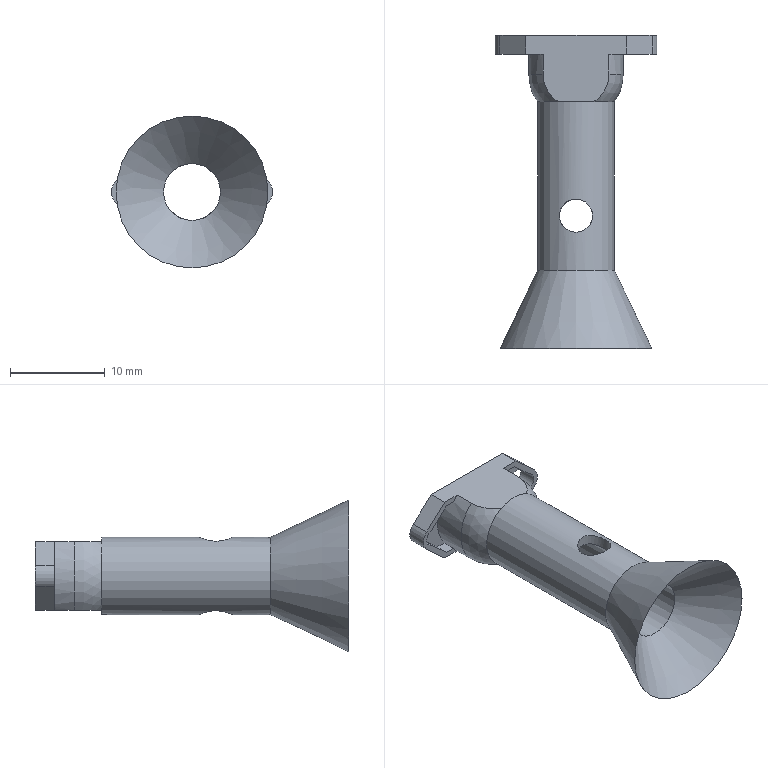Component | NX | AIR_CYLINDER | 1 solid | 36 faces | volume 1058 mm3 | plane 22 | cylinder 10 | sphere 2 | cone 2 | commonest cylinder face diameters 10 x2 3 x2 2 x2 3.5 x2 6 x1 8.13 x1